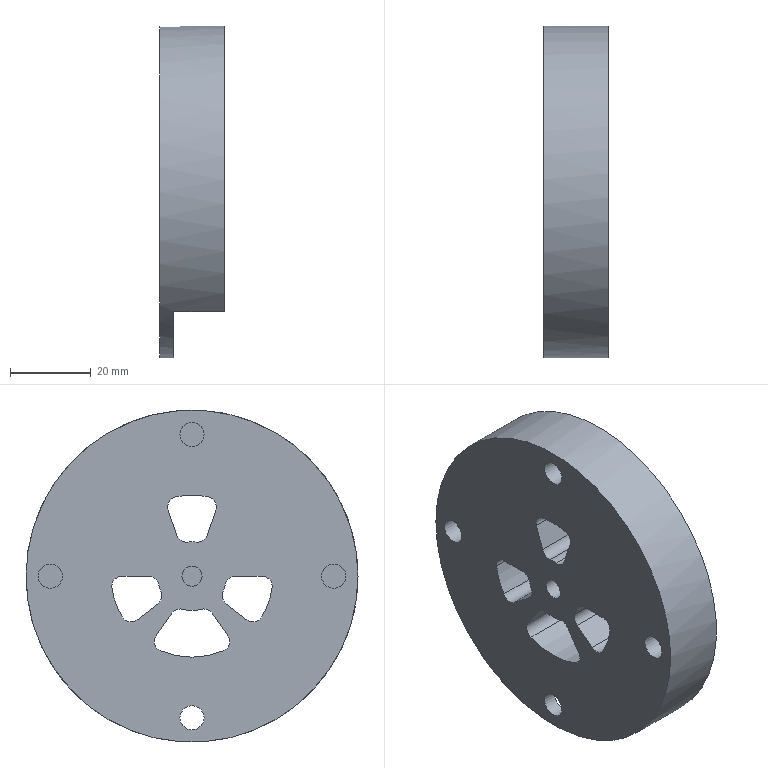Component | NX | OUTER_SUPPORT_PLATE | 1 solid | 50 faces | volume 69497 mm3 | cylinder 32 | plane 18 | commonest cylinder face diameters 5 x17 6 x4 17 x4 40 x4 5.5 x2 82 x1